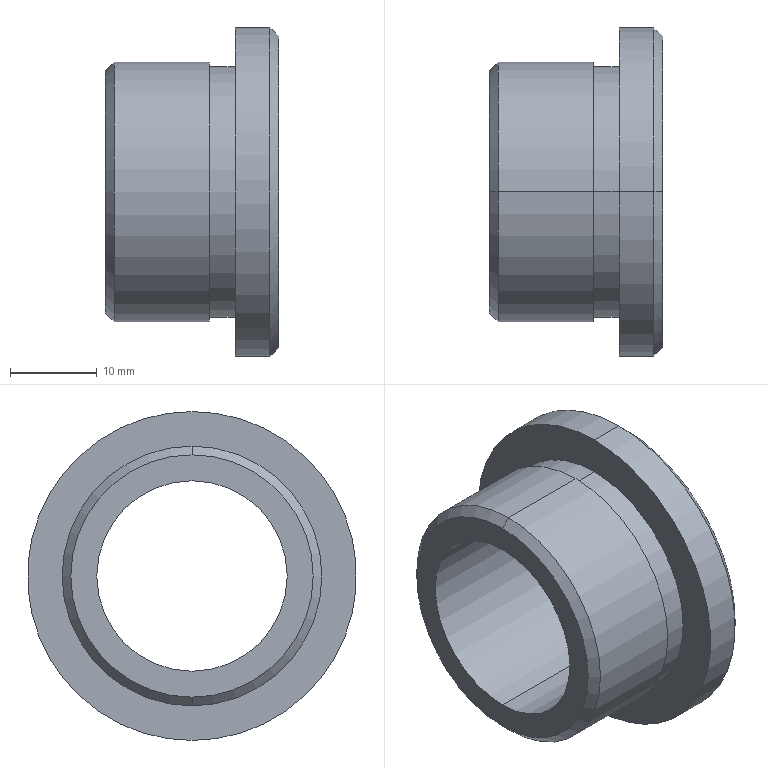Component | SolidWorks | 1CopperSleeve-1 | 1 solid | 16 faces | box 20 x 38 x 38 mm | volume 8427 mm3 | cylinder 8 | cone 4 | plane 4 | commonest cylinder face diameters 22 x2 30 x2 29 x2 38 x2
build123d program:
from build123d import *

# Parameters (mm, degrees)
SKETCH1_R           = 19
BOSS_EXTRUDE1_DEPTH = 5
SKETCH2_R           = 14.5
BOSS_EXTRUDE2_DEPTH = 3
SKETCH3_R           = 15
BOSS_EXTRUDE3_DEPTH = 12
SKETCH4_R           = 11
CUT_EXTRUDE1_DEPTH  = 25
CHAMFER1_SIZE       = 1


with BuildPart() as part:
    # Sketch1 → Boss-Extrude1 (new body)
    with BuildSketch(Plane.XY):
        Circle(SKETCH1_R)
    extrude(amount=BOSS_EXTRUDE1_DEPTH)

    # Sketch2 → Boss-Extrude2 (add)
    with BuildSketch(Plane.XY.offset(5)):
        Circle(SKETCH2_R)
    extrude(amount=BOSS_EXTRUDE2_DEPTH)

    # Sketch3 → Boss-Extrude3 (add)
    with BuildSketch(Plane.XY.offset(8)):
        Circle(SKETCH3_R)
    extrude(amount=BOSS_EXTRUDE3_DEPTH)

    # Sketch4 → Cut-Extrude1 (cut, symmetric)
    with BuildSketch(Plane.XY.offset(20)):
        Circle(SKETCH4_R)
    extrude(amount=CUT_EXTRUDE1_DEPTH, both=True, mode=Mode.SUBTRACT)

    # Chamfer1
    chamfer1_edges = [part.edges().sort_by_distance(p)[0] for p in [
        (-15, 0, 20),
        (-19, 0, 0),
    ]]
    chamfer(chamfer1_edges, length=CHAMFER1_SIZE)


solid = part.part

# Placed as in the assembly
solid = solid.moved(Location((220.5, 65, 0), (0, -90, 0)))
STEP:
#1=CARTESIAN_POINT('',(8.681,2.559,-0.7087));
#2=VERTEX_POINT('',#1);
#3=CARTESIAN_POINT('',(8.681,2.559,0.7087));
#4=VERTEX_POINT('',#3);
#5=CARTESIAN_POINT('',(8.681,2.559,-0.));
#6=DIRECTION('',(1.,-0.,-0.));
#7=DIRECTION('',(0.,0.,1.));
#8=AXIS2_PLACEMENT_3D('',#5,#6,#7);
#9=CIRCLE('',#8,0.7087);
#10=EDGE_CURVE('',#2,#4,#9,.T.);
#11=ORIENTED_EDGE('',*,*,#10,.F.);
#12=CARTESIAN_POINT('',(8.642,2.559,-0.748));
#13=VERTEX_POINT('',#12);
#14=CARTESIAN_POINT('',(8.642,2.559,-0.748));
#15=DIRECTION('',(-0.7071,0.,-0.7071));
#16=VECTOR('',#15,39.37);
#17=LINE('',#14,#16);
#18=EDGE_CURVE('',#2,#13,#17,.T.);
#19=ORIENTED_EDGE('',*,*,#18,.T.);
#20=CARTESIAN_POINT('',(8.642,2.559,0.748));
#21=VERTEX_POINT('',#20);
#22=CARTESIAN_POINT('',(8.642,2.559,-0.));
#23=DIRECTION('',(-1.,0.,0.));
#24=DIRECTION('',(0.,0.,1.));
#25=AXIS2_PLACEMENT_3D('',#22,#23,#24);
#26=CIRCLE('',#25,0.748);
#27=EDGE_CURVE('',#21,#13,#26,.T.);
#28=ORIENTED_EDGE('',*,*,#27,.F.);
#29=CARTESIAN_POINT('',(8.642,2.559,0.748));
#30=DIRECTION('',(-0.7071,0.,0.7071));
#31=VECTOR('',#30,39.37);
#32=LINE('',#29,#31);
#33=EDGE_CURVE('',#4,#21,#32,.T.);
#34=ORIENTED_EDGE('',*,*,#33,.F.);
#35=EDGE_LOOP('',(#11,#19,#28,#34));
#36=FACE_OUTER_BOUND('',#35,.T.);
#37=CARTESIAN_POINT('',(8.642,2.559,-0.));
#38=DIRECTION('',(-1.,0.,0.));
#39=DIRECTION('',(0.,0.,1.));
#40=AXIS2_PLACEMENT_3D('',#37,#38,#39);
#41=CONICAL_SURFACE('',#40,0.748,0.7854);
#42=ADVANCED_FACE('',(#36),#41,.T.);
#43=CARTESIAN_POINT('',(7.894,2.559,0.5512));
#44=VERTEX_POINT('',#43);
#45=CARTESIAN_POINT('',(7.894,2.559,-0.5512));
#46=VERTEX_POINT('',#45);
#47=CARTESIAN_POINT('',(7.894,2.559,-0.));
#48=DIRECTION('',(-1.,0.,0.));
#49=DIRECTION('',(0.,0.,1.));
#50=AXIS2_PLACEMENT_3D('',#47,#48,#49);
#51=CIRCLE('',#50,0.5512);
#52=EDGE_CURVE('',#44,#46,#51,.T.);
#53=ORIENTED_EDGE('',*,*,#52,.F.);
#54=CARTESIAN_POINT('',(7.933,2.559,0.5906));
#55=VERTEX_POINT('',#54);
#56=CARTESIAN_POINT('',(7.894,2.559,0.5512));
#57=DIRECTION('',(0.7071,0.,0.7071));
#58=VECTOR('',#57,39.37);
#59=LINE('',#56,#58);
#60=EDGE_CURVE('',#44,#55,#59,.T.);
#61=ORIENTED_EDGE('',*,*,#60,.T.);
#62=CARTESIAN_POINT('',(7.933,2.559,-0.5906));
#63=VERTEX_POINT('',#62);
#64=CARTESIAN_POINT('',(7.933,2.559,-0.));
#65=DIRECTION('',(1.,-0.,-0.));
#66=DIRECTION('',(0.,0.,1.));
#67=AXIS2_PLACEMENT_3D('',#64,#65,#66);
#68=CIRCLE('',#67,0.5906);
#69=EDGE_CURVE('',#63,#55,#68,.T.);
#70=ORIENTED_EDGE('',*,*,#69,.F.);
#71=CARTESIAN_POINT('',(7.894,2.559,-0.5512));
#72=DIRECTION('',(0.7071,-0.,-0.7071));
#73=VECTOR('',#72,39.37);
#74=LINE('',#71,#73);
#75=EDGE_CURVE('',#46,#63,#74,.T.);
#76=ORIENTED_EDGE('',*,*,#75,.F.);
#77=EDGE_LOOP('',(#53,#61,#70,#76));
#78=FACE_OUTER_BOUND('',#77,.T.);
#79=CARTESIAN_POINT('',(7.894,2.559,-0.));
#80=DIRECTION('',(1.,-0.,-0.));
#81=DIRECTION('',(0.,0.,-1.));
#82=AXIS2_PLACEMENT_3D('',#79,#80,#81);
#83=CONICAL_SURFACE('',#82,0.5512,0.7854);
#84=ADVANCED_FACE('',(#78),#83,.T.);
#85=CARTESIAN_POINT('',(8.681,2.559,-0.4331));
#86=VERTEX_POINT('',#85);
#87=CARTESIAN_POINT('',(8.681,2.559,0.4331));
#88=VERTEX_POINT('',#87);
#89=CARTESIAN_POINT('',(8.681,2.559,-0.));
#90=DIRECTION('',(-1.,0.,0.));
#91=DIRECTION('',(0.,0.,1.));
#92=AXIS2_PLACEMENT_3D('',#89,#90,#91);
#93=CIRCLE('',#92,0.4331);
#94=EDGE_CURVE('',#86,#88,#93,.T.);
#95=ORIENTED_EDGE('',*,*,#94,.F.);
#96=CARTESIAN_POINT('',(7.894,2.559,-0.4331));
#97=VERTEX_POINT('',#96);
#98=CARTESIAN_POINT('',(8.878,2.559,-0.4331));
#99=DIRECTION('',(-1.,0.,0.));
#100=VECTOR('',#99,39.37);
#101=LINE('',#98,#100);
#102=EDGE_CURVE('',#86,#97,#101,.T.);
#103=ORIENTED_EDGE('',*,*,#102,.T.);
#104=CARTESIAN_POINT('',(7.894,2.559,0.4331));
#105=VERTEX_POINT('',#104);
#106=CARTESIAN_POINT('',(7.894,2.559,-0.));
#107=DIRECTION('',(-1.,0.,0.));
#108=DIRECTION('',(0.,0.,1.));
#109=AXIS2_PLACEMENT_3D('',#106,#107,#108);
#110=CIRCLE('',#109,0.4331);
#111=EDGE_CURVE('',#97,#105,#110,.T.);
#112=ORIENTED_EDGE('',*,*,#111,.T.);
#113=CARTESIAN_POINT('',(8.878,2.559,0.4331));
#114=DIRECTION('',(-1.,0.,0.));
#115=VECTOR('',#114,39.37);
#116=LINE('',#113,#115);
#117=EDGE_CURVE('',#88,#105,#116,.T.);
#118=ORIENTED_EDGE('',*,*,#117,.F.);
#119=EDGE_LOOP('',(#95,#103,#112,#118));
#120=FACE_OUTER_BOUND('',#119,.T.);
#121=CARTESIAN_POINT('',(8.878,2.559,-0.));
#122=DIRECTION('',(-1.,0.,0.));
#123=DIRECTION('',(0.,0.,1.));
#124=AXIS2_PLACEMENT_3D('',#121,#122,#123);
#125=CYLINDRICAL_SURFACE('',#124,0.4331);
#126=ADVANCED_FACE('',(#120),#125,.F.);
#127=ORIENTED_EDGE('',*,*,#69,.T.);
#128=CARTESIAN_POINT('',(8.366,2.559,0.5906));
#129=VERTEX_POINT('',#128);
#130=CARTESIAN_POINT('',(7.894,2.559,0.5906));
#131=DIRECTION('',(1.,-0.,-0.));
#132=VECTOR('',#131,39.37);
#133=LINE('',#130,#132);
#134=EDGE_CURVE('',#55,#129,#133,.T.);
#135=ORIENTED_EDGE('',*,*,#134,.T.);
#136=CARTESIAN_POINT('',(8.366,2.559,-0.5906));
#137=VERTEX_POINT('',#136);
#138=CARTESIAN_POINT('',(8.366,2.559,-0.));
#139=DIRECTION('',(-1.,0.,0.));
#140=DIRECTION('',(0.,0.,1.));
#141=AXIS2_PLACEMENT_3D('',#138,#139,#140);
#142=CIRCLE('',#141,0.5906);
#143=EDGE_CURVE('',#129,#137,#142,.T.);
#144=ORIENTED_EDGE('',*,*,#143,.T.);
#145=CARTESIAN_POINT('',(7.894,2.559,-0.5906));
#146=DIRECTION('',(1.,-0.,-0.));
#147=VECTOR('',#146,39.37);
#148=LINE('',#145,#147);
#149=EDGE_CURVE('',#63,#137,#148,.T.);
#150=ORIENTED_EDGE('',*,*,#149,.F.);
#151=EDGE_LOOP('',(#127,#135,#144,#150));
#152=FACE_OUTER_BOUND('',#151,.T.);
#153=CARTESIAN_POINT('',(7.894,2.559,-0.));
#154=DIRECTION('',(1.,-0.,-0.));
#155=DIRECTION('',(0.,0.,-1.));
#156=AXIS2_PLACEMENT_3D('',#153,#154,#155);
#157=CYLINDRICAL_SURFACE('',#156,0.5906);
#158=ADVANCED_FACE('',(#152),#157,.T.);
#159=CARTESIAN_POINT('',(8.366,2.559,0.5709));
#160=VERTEX_POINT('',#159);
#161=CARTESIAN_POINT('',(8.366,2.559,-0.5709));
#162=VERTEX_POINT('',#161);
#163=CARTESIAN_POINT('',(8.366,2.559,-0.));
#164=DIRECTION('',(-1.,0.,0.));
#165=DIRECTION('',(0.,0.,1.));
#166=AXIS2_PLACEMENT_3D('',#163,#164,#165);
#167=CIRCLE('',#166,0.5709);
#168=EDGE_CURVE('',#160,#162,#167,.T.);
#169=ORIENTED_EDGE('',*,*,#168,.F.);
#170=CARTESIAN_POINT('',(8.484,2.559,0.5709));
#171=VERTEX_POINT('',#170);
#172=CARTESIAN_POINT('',(8.366,2.559,0.5709));
#173=DIRECTION('',(1.,-0.,-0.));
#174=VECTOR('',#173,39.37);
#175=LINE('',#172,#174);
#176=EDGE_CURVE('',#160,#171,#175,.T.);
#177=ORIENTED_EDGE('',*,*,#176,.T.);
#178=CARTESIAN_POINT('',(8.484,2.559,-0.5709));
#179=VERTEX_POINT('',#178);
#180=CARTESIAN_POINT('',(8.484,2.559,-0.));
#181=DIRECTION('',(-1.,0.,0.));
#182=DIRECTION('',(0.,0.,1.));
#183=AXIS2_PLACEMENT_3D('',#180,#181,#182);
#184=CIRCLE('',#183,0.5709);
#185=EDGE_CURVE('',#171,#179,#184,.T.);
#186=ORIENTED_EDGE('',*,*,#185,.T.);
#187=CARTESIAN_POINT('',(8.366,2.559,-0.5709));
#188=DIRECTION('',(1.,-0.,-0.));
#189=VECTOR('',#188,39.37);
#190=LINE('',#187,#189);
#191=EDGE_CURVE('',#162,#179,#190,.T.);
#192=ORIENTED_EDGE('',*,*,#191,.F.);
#193=EDGE_LOOP('',(#169,#177,#186,#192));
#194=FACE_OUTER_BOUND('',#193,.T.);
#195=CARTESIAN_POINT('',(8.366,2.559,-0.));
#196=DIRECTION('',(1.,-0.,-0.));
#197=DIRECTION('',(0.,0.,-1.));
#198=AXIS2_PLACEMENT_3D('',#195,#196,#197);
#199=CYLINDRICAL_SURFACE('',#198,0.5709);
#200=ADVANCED_FACE('',(#194),#199,.T.);
#201=CARTESIAN_POINT('',(8.484,2.559,0.748));
#202=VERTEX_POINT('',#201);
#203=CARTESIAN_POINT('',(8.484,2.559,-0.748));
#204=VERTEX_POINT('',#203);
#205=CARTESIAN_POINT('',(8.484,2.559,-0.));
#206=DIRECTION('',(-1.,0.,0.));
#207=DIRECTION('',(0.,0.,1.));
#208=AXIS2_PLACEMENT_3D('',#205,#206,#207);
#209=CIRCLE('',#208,0.748);
#210=EDGE_CURVE('',#202,#204,#209,.T.);
#211=ORIENTED_EDGE('',*,*,#210,.F.);
#212=CARTESIAN_POINT('',(8.484,2.559,0.748));
#213=DIRECTION('',(1.,-0.,-0.));
#214=VECTOR('',#213,39.37);
#215=LINE('',#212,#214);
#216=EDGE_CURVE('',#202,#21,#215,.T.);
#217=ORIENTED_EDGE('',*,*,#216,.T.);
#218=ORIENTED_EDGE('',*,*,#27,.T.);
#219=CARTESIAN_POINT('',(8.484,2.559,-0.748));
#220=DIRECTION('',(1.,-0.,-0.));
#221=VECTOR('',#220,39.37);
#222=LINE('',#219,#221);
#223=EDGE_CURVE('',#204,#13,#222,.T.);
#224=ORIENTED_EDGE('',*,*,#223,.F.);
#225=EDGE_LOOP('',(#211,#217,#218,#224));
#226=FACE_OUTER_BOUND('',#225,.T.);
#227=CARTESIAN_POINT('',(8.484,2.559,-0.));
#228=DIRECTION('',(1.,-0.,-0.));
#229=DIRECTION('',(0.,0.,-1.));
#230=AXIS2_PLACEMENT_3D('',#227,#228,#229);
#231=CYLINDRICAL_SURFACE('',#230,0.748);
#232=ADVANCED_FACE('',(#226),#231,.T.);
#233=ORIENTED_EDGE('',*,*,#216,.F.);
#234=CARTESIAN_POINT('',(8.484,2.559,-0.));
#235=DIRECTION('',(-1.,0.,0.));
#236=DIRECTION('',(0.,0.,1.));
#237=AXIS2_PLACEMENT_3D('',#234,#235,#236);
#238=CIRCLE('',#237,0.748);
#239=EDGE_CURVE('',#204,#202,#238,.T.);
#240=ORIENTED_EDGE('',*,*,#239,.F.);
#241=ORIENTED_EDGE('',*,*,#223,.T.);
#242=CARTESIAN_POINT('',(8.642,2.559,-0.));
#243=DIRECTION('',(-1.,0.,0.));
#244=DIRECTION('',(0.,0.,1.));
#245=AXIS2_PLACEMENT_3D('',#242,#243,#244);
#246=CIRCLE('',#245,0.748);
#247=EDGE_CURVE('',#13,#21,#246,.T.);
#248=ORIENTED_EDGE('',*,*,#247,.T.);
#249=EDGE_LOOP('',(#233,#240,#241,#248));
#250=FACE_OUTER_BOUND('',#249,.T.);
#251=CARTESIAN_POINT('',(8.484,2.559,-0.));
#252=DIRECTION('',(1.,-0.,-0.));
#253=DIRECTION('',(0.,0.,-1.));
#254=AXIS2_PLACEMENT_3D('',#251,#252,#253);
#255=CYLINDRICAL_SURFACE('',#254,0.748);
#256=ADVANCED_FACE('',(#250),#255,.T.);
#257=CARTESIAN_POINT('',(8.484,2.559,-0.));
#258=DIRECTION('',(-1.,0.,0.));
#259=DIRECTION('',(0.,0.,1.));
#260=AXIS2_PLACEMENT_3D('',#257,#258,#259);
#261=CIRCLE('',#260,0.5709);
#262=EDGE_CURVE('',#179,#171,#261,.T.);
#263=ORIENTED_EDGE('',*,*,#262,.F.);
#264=ORIENTED_EDGE('',*,*,#185,.F.);
#265=EDGE_LOOP('',(#263,#264));
#266=FACE_BOUND('',#265,.T.);
#267=ORIENTED_EDGE('',*,*,#239,.T.);
#268=ORIENTED_EDGE('',*,*,#210,.T.);
#269=EDGE_LOOP('',(#267,#268));
#270=FACE_OUTER_BOUND('',#269,.T.);
#271=CARTESIAN_POINT('',(8.484,2.559,-0.));
#272=DIRECTION('',(-1.,0.,0.));
#273=DIRECTION('',(0.,0.,1.));
#274=AXIS2_PLACEMENT_3D('',#271,#272,#273);
#275=PLANE('',#274);
#276=ADVANCED_FACE('',(#266,#270),#275,.T.);
#277=CARTESIAN_POINT('',(8.681,2.559,-0.));
#278=DIRECTION('',(1.,-0.,-0.));
#279=DIRECTION('',(0.,0.,1.));
#280=AXIS2_PLACEMENT_3D('',#277,#278,#279);
#281=CIRCLE('',#280,0.7087);
#282=EDGE_CURVE('',#4,#2,#281,.T.);
#283=ORIENTED_EDGE('',*,*,#282,.T.);
#284=ORIENTED_EDGE('',*,*,#10,.T.);
#285=EDGE_LOOP('',(#283,#284));
#286=FACE_OUTER_BOUND('',#285,.T.);
#287=CARTESIAN_POINT('',(8.681,2.559,-0.));
#288=DIRECTION('',(-1.,0.,0.));
#289=DIRECTION('',(0.,0.,1.));
#290=AXIS2_PLACEMENT_3D('',#287,#288,#289);
#291=CIRCLE('',#290,0.4331);
#292=EDGE_CURVE('',#88,#86,#291,.T.);
#293=ORIENTED_EDGE('',*,*,#292,.T.);
#294=ORIENTED_EDGE('',*,*,#94,.T.);
#295=EDGE_LOOP('',(#293,#294));
#296=FACE_BOUND('',#295,.T.);
#297=CARTESIAN_POINT('',(8.681,2.559,-0.));
#298=DIRECTION('',(-1.,0.,0.));
#299=DIRECTION('',(0.,0.,1.));
#300=AXIS2_PLACEMENT_3D('',#297,#298,#299);
#301=PLANE('',#300);
#302=ADVANCED_FACE('',(#286,#296),#301,.F.);
#303=ORIENTED_EDGE('',*,*,#176,.F.);
#304=CARTESIAN_POINT('',(8.366,2.559,-0.));
#305=DIRECTION('',(-1.,0.,0.));
#306=DIRECTION('',(0.,0.,1.));
#307=AXIS2_PLACEMENT_3D('',#304,#305,#306);
#308=CIRCLE('',#307,0.5709);
#309=EDGE_CURVE('',#162,#160,#308,.T.);
#310=ORIENTED_EDGE('',*,*,#309,.F.);
#311=ORIENTED_EDGE('',*,*,#191,.T.);
#312=ORIENTED_EDGE('',*,*,#262,.T.);
#313=EDGE_LOOP('',(#303,#310,#311,#312));
#314=FACE_OUTER_BOUND('',#313,.T.);
#315=CARTESIAN_POINT('',(8.366,2.559,-0.));
#316=DIRECTION('',(1.,-0.,-0.));
#317=DIRECTION('',(0.,0.,-1.));
#318=AXIS2_PLACEMENT_3D('',#315,#316,#317);
#319=CYLINDRICAL_SURFACE('',#318,0.5709);
#320=ADVANCED_FACE('',(#314),#319,.T.);
#321=ORIENTED_EDGE('',*,*,#134,.F.);
#322=CARTESIAN_POINT('',(7.933,2.559,-0.));
#323=DIRECTION('',(1.,-0.,-0.));
#324=DIRECTION('',(0.,0.,1.));
#325=AXIS2_PLACEMENT_3D('',#322,#323,#324);
#326=CIRCLE('',#325,0.5906);
#327=EDGE_CURVE('',#55,#63,#326,.T.);
#328=ORIENTED_EDGE('',*,*,#327,.T.);
#329=ORIENTED_EDGE('',*,*,#149,.T.);
#330=CARTESIAN_POINT('',(8.366,2.559,-0.));
#331=DIRECTION('',(-1.,0.,0.));
#332=DIRECTION('',(0.,0.,1.));
#333=AXIS2_PLACEMENT_3D('',#330,#331,#332);
#334=CIRCLE('',#333,0.5906);
#335=EDGE_CURVE('',#137,#129,#334,.T.);
#336=ORIENTED_EDGE('',*,*,#335,.T.);
#337=EDGE_LOOP('',(#321,#328,#329,#336));
#338=FACE_OUTER_BOUND('',#337,.T.);
#339=CARTESIAN_POINT('',(7.894,2.559,-0.));
#340=DIRECTION('',(1.,-0.,-0.));
#341=DIRECTION('',(0.,0.,-1.));
#342=AXIS2_PLACEMENT_3D('',#339,#340,#341);
#343=CYLINDRICAL_SURFACE('',#342,0.5906);
#344=ADVANCED_FACE('',(#338),#343,.T.);
#345=CARTESIAN_POINT('',(7.894,2.559,-0.));
#346=DIRECTION('',(-1.,0.,0.));
#347=DIRECTION('',(0.,0.,1.));
#348=AXIS2_PLACEMENT_3D('',#345,#346,#347);
#349=CIRCLE('',#348,0.5512);
#350=EDGE_CURVE('',#46,#44,#349,.T.);
#351=ORIENTED_EDGE('',*,*,#350,.T.);
#352=ORIENTED_EDGE('',*,*,#52,.T.);
#353=EDGE_LOOP('',(#351,#352));
#354=FACE_OUTER_BOUND('',#353,.T.);
#355=CARTESIAN_POINT('',(7.894,2.559,-0.));
#356=DIRECTION('',(-1.,0.,0.));
#357=DIRECTION('',(0.,0.,1.));
#358=AXIS2_PLACEMENT_3D('',#355,#356,#357);
#359=CIRCLE('',#358,0.4331);
#360=EDGE_CURVE('',#105,#97,#359,.T.);
#361=ORIENTED_EDGE('',*,*,#360,.F.);
#362=ORIENTED_EDGE('',*,*,#111,.F.);
#363=EDGE_LOOP('',(#361,#362));
#364=FACE_BOUND('',#363,.T.);
#365=CARTESIAN_POINT('',(7.894,2.559,-0.));
#366=DIRECTION('',(-1.,0.,0.));
#367=DIRECTION('',(0.,0.,1.));
#368=AXIS2_PLACEMENT_3D('',#365,#366,#367);
#369=PLANE('',#368);
#370=ADVANCED_FACE('',(#354,#364),#369,.T.);
#371=ORIENTED_EDGE('',*,*,#309,.T.);
#372=ORIENTED_EDGE('',*,*,#168,.T.);
#373=EDGE_LOOP('',(#371,#372));
#374=FACE_BOUND('',#373,.T.);
#375=ORIENTED_EDGE('',*,*,#335,.F.);
#376=ORIENTED_EDGE('',*,*,#143,.F.);
#377=EDGE_LOOP('',(#375,#376));
#378=FACE_OUTER_BOUND('',#377,.T.);
#379=CARTESIAN_POINT('',(8.366,2.559,-0.));
#380=DIRECTION('',(-1.,0.,0.));
#381=DIRECTION('',(0.,0.,1.));
#382=AXIS2_PLACEMENT_3D('',#379,#380,#381);
#383=PLANE('',#382);
#384=ADVANCED_FACE('',(#374,#378),#383,.F.);
#385=ORIENTED_EDGE('',*,*,#102,.F.);
#386=ORIENTED_EDGE('',*,*,#292,.F.);
#387=ORIENTED_EDGE('',*,*,#117,.T.);
#388=ORIENTED_EDGE('',*,*,#360,.T.);
#389=EDGE_LOOP('',(#385,#386,#387,#388));
#390=FACE_OUTER_BOUND('',#389,.T.);
#391=CARTESIAN_POINT('',(8.878,2.559,-0.));
#392=DIRECTION('',(-1.,0.,0.));
#393=DIRECTION('',(0.,0.,1.));
#394=AXIS2_PLACEMENT_3D('',#391,#392,#393);
#395=CYLINDRICAL_SURFACE('',#394,0.4331);
#396=ADVANCED_FACE('',(#390),#395,.F.);
#397=ORIENTED_EDGE('',*,*,#60,.F.);
#398=ORIENTED_EDGE('',*,*,#350,.F.);
#399=ORIENTED_EDGE('',*,*,#75,.T.);
#400=ORIENTED_EDGE('',*,*,#327,.F.);
#401=EDGE_LOOP('',(#397,#398,#399,#400));
#402=FACE_OUTER_BOUND('',#401,.T.);
#403=CARTESIAN_POINT('',(7.894,2.559,-0.));
#404=DIRECTION('',(1.,-0.,-0.));
#405=DIRECTION('',(0.,0.,-1.));
#406=AXIS2_PLACEMENT_3D('',#403,#404,#405);
#407=CONICAL_SURFACE('',#406,0.5512,0.7854);
#408=ADVANCED_FACE('',(#402),#407,.T.);
#409=ORIENTED_EDGE('',*,*,#18,.F.);
#410=ORIENTED_EDGE('',*,*,#282,.F.);
#411=ORIENTED_EDGE('',*,*,#33,.T.);
#412=ORIENTED_EDGE('',*,*,#247,.F.);
#413=EDGE_LOOP('',(#409,#410,#411,#412));
#414=FACE_OUTER_BOUND('',#413,.T.);
#415=CARTESIAN_POINT('',(8.642,2.559,-0.));
#416=DIRECTION('',(-1.,0.,0.));
#417=DIRECTION('',(0.,0.,1.));
#418=AXIS2_PLACEMENT_3D('',#415,#416,#417);
#419=CONICAL_SURFACE('',#418,0.748,0.7854);
#420=ADVANCED_FACE('',(#414),#419,.T.);
#421=CLOSED_SHELL('',(#42,#84,#126,#158,#200,#232,#256,#276,#302,#320,#344,#370,#384,#396,#408,#420));
#422=MANIFOLD_SOLID_BREP('',#421);
#423=CARTESIAN_POINT('',(0.,0.,0.));
#424=DIRECTION('',(0.,0.,1.));
#425=DIRECTION('',(1.,0.,0.));
#426=AXIS2_PLACEMENT_3D('',#423,#424,#425);
#427=(LENGTH_UNIT()NAMED_UNIT(*)SI_UNIT($,.METRE.));
#428=LENGTH_MEASURE_WITH_UNIT(LENGTH_MEASURE(0.0254),#427);
#429=DIMENSIONAL_EXPONENTS(1.,0.,0.,0.,0.,0.,0.);
#430=(CONVERSION_BASED_UNIT('',#428)LENGTH_UNIT()NAMED_UNIT(#429));
#431=UNCERTAINTY_MEASURE_WITH_UNIT(LENGTH_MEASURE(0.00001),#430,'','');
#432=(NAMED_UNIT(*)PLANE_ANGLE_UNIT()SI_UNIT($,.RADIAN.));
#433=(NAMED_UNIT(*)SI_UNIT($,.STERADIAN.)SOLID_ANGLE_UNIT());
#434=(GEOMETRIC_REPRESENTATION_CONTEXT(3)GLOBAL_UNCERTAINTY_ASSIGNED_CONTEXT((#431))GLOBAL_UNIT_ASSIGNED_CONTEXT((#430,#432,#433))REPRESENTATION_CONTEXT('',''));
#435=ADVANCED_BREP_SHAPE_REPRESENTATION('',(#422,#426),#434);
#436=COLOUR_RGB('',0.7922,0.8196,0.9333);
#437=FILL_AREA_STYLE_COLOUR('',#436);
#438=FILL_AREA_STYLE('',(#437));
#439=SURFACE_STYLE_FILL_AREA(#438);
#440=SURFACE_SIDE_STYLE('',(#439));
#441=SURFACE_STYLE_USAGE(.BOTH.,#440);
#442=PRESENTATION_STYLE_ASSIGNMENT((#441));
#443=STYLED_ITEM('',(#442),#422);
#444=(LENGTH_UNIT()NAMED_UNIT(*)SI_UNIT($,.METRE.));
#445=LENGTH_MEASURE_WITH_UNIT(LENGTH_MEASURE(0.0254),#444);
#446=DIMENSIONAL_EXPONENTS(1.,0.,0.,0.,0.,0.,0.);
#447=(CONVERSION_BASED_UNIT('',#445)LENGTH_UNIT()NAMED_UNIT(#446));
#448=UNCERTAINTY_MEASURE_WITH_UNIT(LENGTH_MEASURE(0.00001),#447,'','');
#449=(NAMED_UNIT(*)PLANE_ANGLE_UNIT()SI_UNIT($,.RADIAN.));
#450=(NAMED_UNIT(*)SI_UNIT($,.STERADIAN.)SOLID_ANGLE_UNIT());
#451=(GEOMETRIC_REPRESENTATION_CONTEXT(3)GLOBAL_UNCERTAINTY_ASSIGNED_CONTEXT((#448))GLOBAL_UNIT_ASSIGNED_CONTEXT((#447,#449,#450))REPRESENTATION_CONTEXT('',''));
#452=MECHANICAL_DESIGN_GEOMETRIC_PRESENTATION_REPRESENTATION('',(#443),#451);
#453=PRESENTATION_LAYER_ASSIGNMENT('','',(#443));